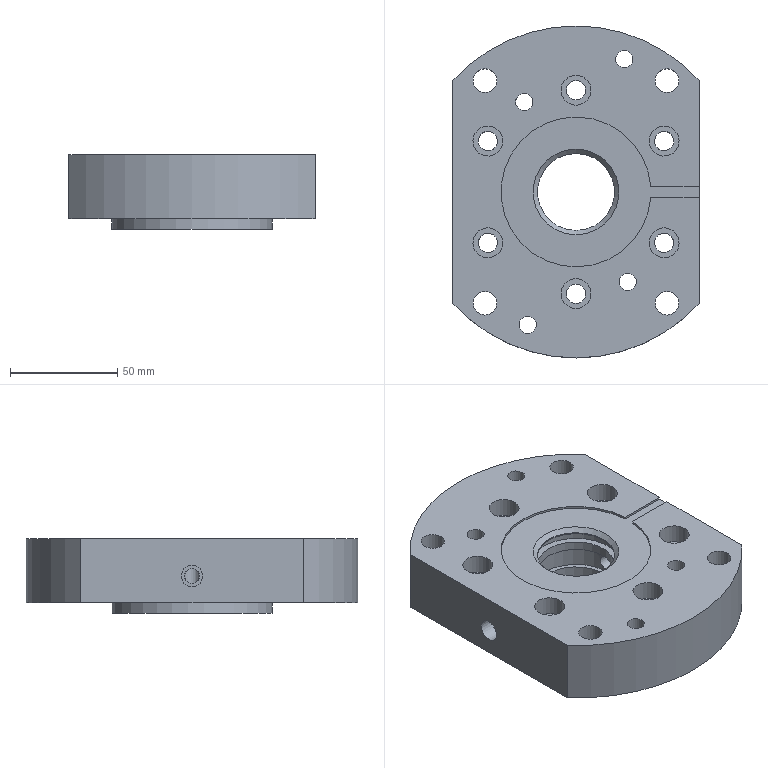Component | NX | FRONT_COVER | 1 solid | 63 faces | volume 415524 mm3 | cylinder 37 | plane 24 | cone 2 | commonest cylinder face diameters 14 x6 9 x6 11 x4 8 x4 17 x4 7 x3 36 x3 155 x2